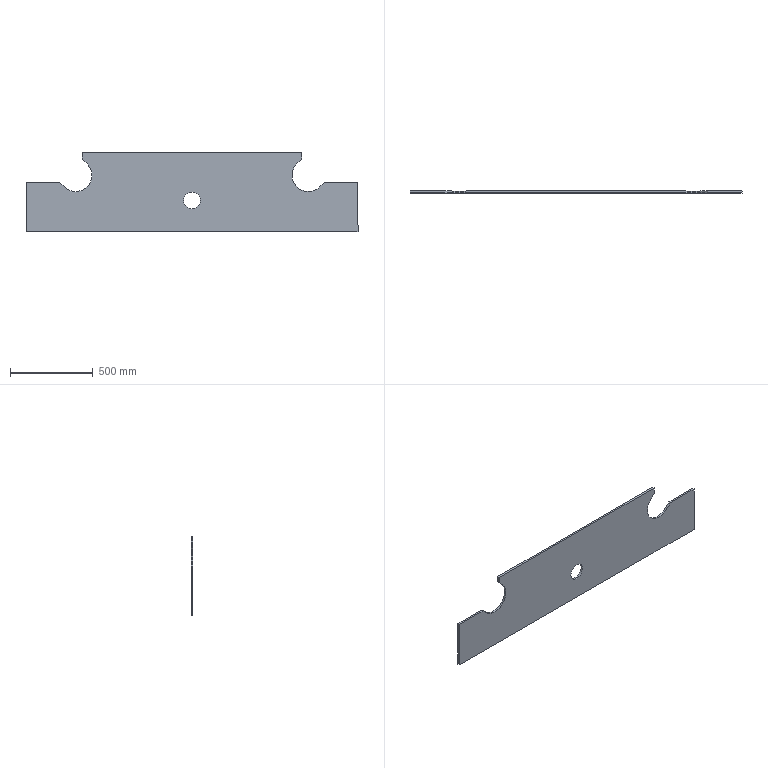Component | SolidWorks | SidePlate-2 | 1 solid | 19 faces | box 2000 x 12 x 476 mm | volume 9555406 mm3 | plane 14 | cylinder 5 | commonest cylinder face diameters 195 x3 100 x2 | material Plain Carbon Steel
STEP:
#1=COLOUR_RGB('',0.7922,0.8196,0.9333);
#2=FILL_AREA_STYLE_COLOUR('',#1);
#3=FILL_AREA_STYLE('',(#2));
#4=SURFACE_STYLE_FILL_AREA(#3);
#5=SURFACE_SIDE_STYLE('',(#4));
#6=SURFACE_STYLE_USAGE(.BOTH.,#5);
#7=PRESENTATION_STYLE_ASSIGNMENT((#6));
#8=CARTESIAN_POINT('',(51.204,45.014,72.956));
#9=VERTEX_POINT('',#8);
#10=CARTESIAN_POINT('',(47.267,45.014,72.956));
#11=VERTEX_POINT('',#10);
#12=CARTESIAN_POINT('',(49.235,45.014,72.956));
#13=DIRECTION('',(-0.,-1.,-0.));
#14=DIRECTION('',(-1.,0.,-0.));
#15=AXIS2_PLACEMENT_3D('',#12,#13,#14);
#16=CIRCLE('',#15,1.969);
#17=EDGE_CURVE('',#9,#11,#16,.T.);
#18=ORIENTED_EDGE('',*,*,#17,.F.);
#19=CARTESIAN_POINT('',(51.204,44.541,72.956));
#20=VERTEX_POINT('',#19);
#21=CARTESIAN_POINT('',(51.204,45.014,72.956));
#22=DIRECTION('',(-0.,-1.,-0.));
#23=VECTOR('',#22,39.37);
#24=LINE('',#21,#23);
#25=EDGE_CURVE('',#9,#20,#24,.T.);
#26=ORIENTED_EDGE('',*,*,#25,.T.);
#27=CARTESIAN_POINT('',(47.267,44.541,72.956));
#28=VERTEX_POINT('',#27);
#29=CARTESIAN_POINT('',(49.235,44.541,72.956));
#30=DIRECTION('',(-0.,-1.,-0.));
#31=DIRECTION('',(-1.,0.,-0.));
#32=AXIS2_PLACEMENT_3D('',#29,#30,#31);
#33=CIRCLE('',#32,1.969);
#34=EDGE_CURVE('',#20,#28,#33,.T.);
#35=ORIENTED_EDGE('',*,*,#34,.T.);
#36=CARTESIAN_POINT('',(47.267,45.014,72.956));
#37=DIRECTION('',(-0.,-1.,-0.));
#38=VECTOR('',#37,39.37);
#39=LINE('',#36,#38);
#40=EDGE_CURVE('',#11,#28,#39,.T.);
#41=ORIENTED_EDGE('',*,*,#40,.F.);
#42=EDGE_LOOP('',(#18,#26,#35,#41));
#43=FACE_OUTER_BOUND('',#42,.T.);
#44=CARTESIAN_POINT('',(49.235,45.014,72.956));
#45=DIRECTION('',(-0.,-1.,-0.));
#46=DIRECTION('',(-1.,0.,-0.));
#47=AXIS2_PLACEMENT_3D('',#44,#45,#46);
#48=CYLINDRICAL_SURFACE('',#47,1.969);
#49=ADVANCED_FACE('',(#43),#48,.F.);
#50=CARTESIAN_POINT('',(79.503,45.014,76.142));
#51=VERTEX_POINT('',#50);
#52=CARTESIAN_POINT('',(72.956,45.014,78.862));
#53=VERTEX_POINT('',#52);
#54=CARTESIAN_POINT('',(76.794,45.014,78.862));
#55=DIRECTION('',(0.,1.,0.));
#56=DIRECTION('',(1.,-0.,0.));
#57=AXIS2_PLACEMENT_3D('',#54,#55,#56);
#58=CIRCLE('',#57,3.839);
#59=EDGE_CURVE('',#51,#53,#58,.T.);
#60=ORIENTED_EDGE('',*,*,#59,.T.);
#61=CARTESIAN_POINT('',(72.956,44.541,78.862));
#62=VERTEX_POINT('',#61);
#63=CARTESIAN_POINT('',(72.956,45.014,78.862));
#64=DIRECTION('',(-0.,-1.,-0.));
#65=VECTOR('',#64,39.37);
#66=LINE('',#63,#65);
#67=EDGE_CURVE('',#53,#62,#66,.T.);
#68=ORIENTED_EDGE('',*,*,#67,.T.);
#69=CARTESIAN_POINT('',(79.503,44.541,76.142));
#70=VERTEX_POINT('',#69);
#71=CARTESIAN_POINT('',(76.794,44.541,78.862));
#72=DIRECTION('',(0.,1.,0.));
#73=DIRECTION('',(1.,-0.,0.));
#74=AXIS2_PLACEMENT_3D('',#71,#72,#73);
#75=CIRCLE('',#74,3.839);
#76=EDGE_CURVE('',#70,#62,#75,.T.);
#77=ORIENTED_EDGE('',*,*,#76,.F.);
#78=CARTESIAN_POINT('',(79.503,45.014,76.142));
#79=DIRECTION('',(-0.,-1.,-0.));
#80=VECTOR('',#79,39.37);
#81=LINE('',#78,#80);
#82=EDGE_CURVE('',#51,#70,#81,.T.);
#83=ORIENTED_EDGE('',*,*,#82,.F.);
#84=EDGE_LOOP('',(#60,#68,#77,#83));
#85=FACE_OUTER_BOUND('',#84,.T.);
#86=CARTESIAN_POINT('',(76.794,45.014,78.862));
#87=DIRECTION('',(-0.,-1.,-0.));
#88=DIRECTION('',(-1.,0.,-0.));
#89=AXIS2_PLACEMENT_3D('',#86,#87,#88);
#90=CYLINDRICAL_SURFACE('',#89,3.839);
#91=ADVANCED_FACE('',(#85),#90,.F.);
#92=CARTESIAN_POINT('',(88.605,44.541,65.555));
#93=VERTEX_POINT('',#92);
#94=CARTESIAN_POINT('',(88.605,44.541,77.287));
#95=VERTEX_POINT('',#94);
#96=CARTESIAN_POINT('',(88.605,44.541,65.555));
#97=DIRECTION('',(-0.,-0.,1.));
#98=VECTOR('',#97,39.37);
#99=LINE('',#96,#98);
#100=EDGE_CURVE('',#93,#95,#99,.T.);
#101=ORIENTED_EDGE('',*,*,#100,.F.);
#102=CARTESIAN_POINT('',(88.605,45.014,65.555));
#103=VERTEX_POINT('',#102);
#104=CARTESIAN_POINT('',(88.605,45.014,65.555));
#105=DIRECTION('',(-0.,-1.,-0.));
#106=VECTOR('',#105,39.37);
#107=LINE('',#104,#106);
#108=EDGE_CURVE('',#103,#93,#107,.T.);
#109=ORIENTED_EDGE('',*,*,#108,.F.);
#110=CARTESIAN_POINT('',(88.605,45.014,77.287));
#111=VERTEX_POINT('',#110);
#112=CARTESIAN_POINT('',(88.605,45.014,65.555));
#113=DIRECTION('',(-0.,-0.,1.));
#114=VECTOR('',#113,39.37);
#115=LINE('',#112,#114);
#116=EDGE_CURVE('',#103,#111,#115,.T.);
#117=ORIENTED_EDGE('',*,*,#116,.T.);
#118=CARTESIAN_POINT('',(88.605,45.014,77.287));
#119=DIRECTION('',(-0.,-1.,-0.));
#120=VECTOR('',#119,39.37);
#121=LINE('',#118,#120);
#122=EDGE_CURVE('',#111,#95,#121,.T.);
#123=ORIENTED_EDGE('',*,*,#122,.T.);
#124=EDGE_LOOP('',(#101,#109,#117,#123));
#125=FACE_OUTER_BOUND('',#124,.T.);
#126=CARTESIAN_POINT('',(88.605,45.014,65.555));
#127=DIRECTION('',(1.,-0.,0.));
#128=DIRECTION('',(-0.,-0.,1.));
#129=AXIS2_PLACEMENT_3D('',#126,#127,#128);
#130=PLANE('',#129);
#131=ADVANCED_FACE('',(#125),#130,.T.);
#132=CARTESIAN_POINT('',(9.865,44.541,65.555));
#133=VERTEX_POINT('',#132);
#134=CARTESIAN_POINT('',(88.605,44.541,65.555));
#135=DIRECTION('',(1.,-0.,0.));
#136=VECTOR('',#135,39.37);
#137=LINE('',#134,#136);
#138=EDGE_CURVE('',#133,#93,#137,.T.);
#139=ORIENTED_EDGE('',*,*,#138,.F.);
#140=CARTESIAN_POINT('',(9.865,45.014,65.555));
#141=VERTEX_POINT('',#140);
#142=CARTESIAN_POINT('',(9.865,45.014,65.555));
#143=DIRECTION('',(-0.,-1.,-0.));
#144=VECTOR('',#143,39.37);
#145=LINE('',#142,#144);
#146=EDGE_CURVE('',#141,#133,#145,.T.);
#147=ORIENTED_EDGE('',*,*,#146,.F.);
#148=CARTESIAN_POINT('',(88.605,45.014,65.555));
#149=DIRECTION('',(1.,-0.,0.));
#150=VECTOR('',#149,39.37);
#151=LINE('',#148,#150);
#152=EDGE_CURVE('',#141,#103,#151,.T.);
#153=ORIENTED_EDGE('',*,*,#152,.T.);
#154=ORIENTED_EDGE('',*,*,#108,.T.);
#155=EDGE_LOOP('',(#139,#147,#153,#154));
#156=FACE_OUTER_BOUND('',#155,.T.);
#157=CARTESIAN_POINT('',(88.605,45.014,65.555));
#158=DIRECTION('',(0.,0.,-1.));
#159=DIRECTION('',(1.,-0.,0.));
#160=AXIS2_PLACEMENT_3D('',#157,#158,#159);
#161=PLANE('',#160);
#162=ADVANCED_FACE('',(#156),#161,.T.);
#163=CARTESIAN_POINT('',(9.865,44.541,77.287));
#164=VERTEX_POINT('',#163);
#165=CARTESIAN_POINT('',(9.865,44.541,65.555));
#166=DIRECTION('',(0.,0.,-1.));
#167=VECTOR('',#166,39.37);
#168=LINE('',#165,#167);
#169=EDGE_CURVE('',#164,#133,#168,.T.);
#170=ORIENTED_EDGE('',*,*,#169,.F.);
#171=CARTESIAN_POINT('',(9.865,45.014,77.287));
#172=VERTEX_POINT('',#171);
#173=CARTESIAN_POINT('',(9.865,45.014,77.287));
#174=DIRECTION('',(-0.,-1.,-0.));
#175=VECTOR('',#174,39.37);
#176=LINE('',#173,#175);
#177=EDGE_CURVE('',#172,#164,#176,.T.);
#178=ORIENTED_EDGE('',*,*,#177,.F.);
#179=CARTESIAN_POINT('',(9.865,45.014,65.555));
#180=DIRECTION('',(0.,0.,-1.));
#181=VECTOR('',#180,39.37);
#182=LINE('',#179,#181);
#183=EDGE_CURVE('',#172,#141,#182,.T.);
#184=ORIENTED_EDGE('',*,*,#183,.T.);
#185=ORIENTED_EDGE('',*,*,#146,.T.);
#186=EDGE_LOOP('',(#170,#178,#184,#185));
#187=FACE_OUTER_BOUND('',#186,.T.);
#188=CARTESIAN_POINT('',(9.865,45.014,65.555));
#189=DIRECTION('',(-1.,0.,-0.));
#190=DIRECTION('',(0.,0.,-1.));
#191=AXIS2_PLACEMENT_3D('',#188,#189,#190);
#192=PLANE('',#191);
#193=ADVANCED_FACE('',(#187),#192,.T.);
#194=CARTESIAN_POINT('',(17.818,44.541,77.287));
#195=VERTEX_POINT('',#194);
#196=CARTESIAN_POINT('',(9.865,44.541,77.287));
#197=DIRECTION('',(-1.,0.,-0.));
#198=VECTOR('',#197,39.37);
#199=LINE('',#196,#198);
#200=EDGE_CURVE('',#195,#164,#199,.T.);
#201=ORIENTED_EDGE('',*,*,#200,.F.);
#202=CARTESIAN_POINT('',(17.818,45.014,77.287));
#203=VERTEX_POINT('',#202);
#204=CARTESIAN_POINT('',(17.818,45.014,77.287));
#205=DIRECTION('',(-0.,-1.,-0.));
#206=VECTOR('',#205,39.37);
#207=LINE('',#204,#206);
#208=EDGE_CURVE('',#203,#195,#207,.T.);
#209=ORIENTED_EDGE('',*,*,#208,.F.);
#210=CARTESIAN_POINT('',(9.865,45.014,77.287));
#211=DIRECTION('',(-1.,0.,-0.));
#212=VECTOR('',#211,39.37);
#213=LINE('',#210,#212);
#214=EDGE_CURVE('',#203,#172,#213,.T.);
#215=ORIENTED_EDGE('',*,*,#214,.T.);
#216=ORIENTED_EDGE('',*,*,#177,.T.);
#217=EDGE_LOOP('',(#201,#209,#215,#216));
#218=FACE_OUTER_BOUND('',#217,.T.);
#219=CARTESIAN_POINT('',(9.865,45.014,77.287));
#220=DIRECTION('',(-0.,-0.,1.));
#221=DIRECTION('',(-1.,0.,-0.));
#222=AXIS2_PLACEMENT_3D('',#219,#220,#221);
#223=PLANE('',#222);
#224=ADVANCED_FACE('',(#218),#223,.T.);
#225=CARTESIAN_POINT('',(18.967,44.541,76.142));
#226=VERTEX_POINT('',#225);
#227=CARTESIAN_POINT('',(17.818,44.541,77.287));
#228=DIRECTION('',(-0.7085,-0.,0.7057));
#229=VECTOR('',#228,39.37);
#230=LINE('',#227,#229);
#231=EDGE_CURVE('',#226,#195,#230,.T.);
#232=ORIENTED_EDGE('',*,*,#231,.F.);
#233=CARTESIAN_POINT('',(18.967,45.014,76.142));
#234=VERTEX_POINT('',#233);
#235=CARTESIAN_POINT('',(18.967,45.014,76.142));
#236=DIRECTION('',(-0.,-1.,-0.));
#237=VECTOR('',#236,39.37);
#238=LINE('',#235,#237);
#239=EDGE_CURVE('',#234,#226,#238,.T.);
#240=ORIENTED_EDGE('',*,*,#239,.F.);
#241=CARTESIAN_POINT('',(17.818,45.014,77.287));
#242=DIRECTION('',(-0.7085,-0.,0.7057));
#243=VECTOR('',#242,39.37);
#244=LINE('',#241,#243);
#245=EDGE_CURVE('',#234,#203,#244,.T.);
#246=ORIENTED_EDGE('',*,*,#245,.T.);
#247=ORIENTED_EDGE('',*,*,#208,.T.);
#248=EDGE_LOOP('',(#232,#240,#246,#247));
#249=FACE_OUTER_BOUND('',#248,.T.);
#250=CARTESIAN_POINT('',(17.818,45.014,77.287));
#251=DIRECTION('',(0.7057,-0.,0.7085));
#252=DIRECTION('',(-0.7085,-0.,0.7057));
#253=AXIS2_PLACEMENT_3D('',#250,#251,#252);
#254=PLANE('',#253);
#255=ADVANCED_FACE('',(#249),#254,.T.);
#256=CARTESIAN_POINT('',(24.396,44.541,81.571));
#257=VERTEX_POINT('',#256);
#258=CARTESIAN_POINT('',(21.676,44.541,78.862));
#259=DIRECTION('',(0.,1.,0.));
#260=DIRECTION('',(-1.,0.,-0.));
#261=AXIS2_PLACEMENT_3D('',#258,#259,#260);
#262=CIRCLE('',#261,3.839);
#263=EDGE_CURVE('',#257,#226,#262,.T.);
#264=ORIENTED_EDGE('',*,*,#263,.F.);
#265=CARTESIAN_POINT('',(24.396,45.014,81.571));
#266=VERTEX_POINT('',#265);
#267=CARTESIAN_POINT('',(24.396,45.014,81.571));
#268=DIRECTION('',(-0.,-1.,-0.));
#269=VECTOR('',#268,39.37);
#270=LINE('',#267,#269);
#271=EDGE_CURVE('',#266,#257,#270,.T.);
#272=ORIENTED_EDGE('',*,*,#271,.F.);
#273=CARTESIAN_POINT('',(21.676,45.014,78.862));
#274=DIRECTION('',(0.,1.,0.));
#275=DIRECTION('',(-1.,0.,-0.));
#276=AXIS2_PLACEMENT_3D('',#273,#274,#275);
#277=CIRCLE('',#276,3.839);
#278=EDGE_CURVE('',#266,#234,#277,.T.);
#279=ORIENTED_EDGE('',*,*,#278,.T.);
#280=ORIENTED_EDGE('',*,*,#239,.T.);
#281=EDGE_LOOP('',(#264,#272,#279,#280));
#282=FACE_OUTER_BOUND('',#281,.T.);
#283=CARTESIAN_POINT('',(21.676,45.014,78.862));
#284=DIRECTION('',(-0.,-1.,-0.));
#285=DIRECTION('',(-1.,0.,-0.));
#286=AXIS2_PLACEMENT_3D('',#283,#284,#285);
#287=CYLINDRICAL_SURFACE('',#286,3.839);
#288=ADVANCED_FACE('',(#282),#287,.F.);
#289=CARTESIAN_POINT('',(23.251,44.541,82.72));
#290=VERTEX_POINT('',#289);
#291=CARTESIAN_POINT('',(23.251,44.541,82.72));
#292=DIRECTION('',(0.7057,0.,-0.7085));
#293=VECTOR('',#292,39.37);
#294=LINE('',#291,#293);
#295=EDGE_CURVE('',#290,#257,#294,.T.);
#296=ORIENTED_EDGE('',*,*,#295,.F.);
#297=CARTESIAN_POINT('',(23.251,45.014,82.72));
#298=VERTEX_POINT('',#297);
#299=CARTESIAN_POINT('',(23.251,45.014,82.72));
#300=DIRECTION('',(-0.,-1.,-0.));
#301=VECTOR('',#300,39.37);
#302=LINE('',#299,#301);
#303=EDGE_CURVE('',#298,#290,#302,.T.);
#304=ORIENTED_EDGE('',*,*,#303,.F.);
#305=CARTESIAN_POINT('',(23.251,45.014,82.72));
#306=DIRECTION('',(0.7057,0.,-0.7085));
#307=VECTOR('',#306,39.37);
#308=LINE('',#305,#307);
#309=EDGE_CURVE('',#298,#266,#308,.T.);
#310=ORIENTED_EDGE('',*,*,#309,.T.);
#311=ORIENTED_EDGE('',*,*,#271,.T.);
#312=EDGE_LOOP('',(#296,#304,#310,#311));
#313=FACE_OUTER_BOUND('',#312,.T.);
#314=CARTESIAN_POINT('',(23.251,45.014,82.72));
#315=DIRECTION('',(-0.7085,0.,-0.7057));
#316=DIRECTION('',(0.7057,0.,-0.7085));
#317=AXIS2_PLACEMENT_3D('',#314,#315,#316);
#318=PLANE('',#317);
#319=ADVANCED_FACE('',(#313),#318,.T.);
#320=CARTESIAN_POINT('',(23.251,44.541,84.295));
#321=VERTEX_POINT('',#320);
#322=CARTESIAN_POINT('',(23.251,44.541,84.295));
#323=DIRECTION('',(0.,0.,-1.));
#324=VECTOR('',#323,39.37);
#325=LINE('',#322,#324);
#326=EDGE_CURVE('',#321,#290,#325,.T.);
#327=ORIENTED_EDGE('',*,*,#326,.F.);
#328=CARTESIAN_POINT('',(23.251,45.014,84.295));
#329=VERTEX_POINT('',#328);
#330=CARTESIAN_POINT('',(23.251,45.014,84.295));
#331=DIRECTION('',(-0.,-1.,-0.));
#332=VECTOR('',#331,39.37);
#333=LINE('',#330,#332);
#334=EDGE_CURVE('',#329,#321,#333,.T.);
#335=ORIENTED_EDGE('',*,*,#334,.F.);
#336=CARTESIAN_POINT('',(23.251,45.014,84.295));
#337=DIRECTION('',(0.,0.,-1.));
#338=VECTOR('',#337,39.37);
#339=LINE('',#336,#338);
#340=EDGE_CURVE('',#329,#298,#339,.T.);
#341=ORIENTED_EDGE('',*,*,#340,.T.);
#342=ORIENTED_EDGE('',*,*,#303,.T.);
#343=EDGE_LOOP('',(#327,#335,#341,#342));
#344=FACE_OUTER_BOUND('',#343,.T.);
#345=CARTESIAN_POINT('',(23.251,45.014,84.295));
#346=DIRECTION('',(-1.,0.,-0.));
#347=DIRECTION('',(0.,0.,-1.));
#348=AXIS2_PLACEMENT_3D('',#345,#346,#347);
#349=PLANE('',#348);
#350=ADVANCED_FACE('',(#344),#349,.T.);
#351=CARTESIAN_POINT('',(75.22,44.541,84.295));
#352=VERTEX_POINT('',#351);
#353=CARTESIAN_POINT('',(75.22,44.541,84.295));
#354=DIRECTION('',(-1.,0.,-0.));
#355=VECTOR('',#354,39.37);
#356=LINE('',#353,#355);
#357=EDGE_CURVE('',#352,#321,#356,.T.);
#358=ORIENTED_EDGE('',*,*,#357,.F.);
#359=CARTESIAN_POINT('',(75.22,45.014,84.295));
#360=VERTEX_POINT('',#359);
#361=CARTESIAN_POINT('',(75.22,45.014,84.295));
#362=DIRECTION('',(-0.,-1.,-0.));
#363=VECTOR('',#362,39.37);
#364=LINE('',#361,#363);
#365=EDGE_CURVE('',#360,#352,#364,.T.);
#366=ORIENTED_EDGE('',*,*,#365,.F.);
#367=CARTESIAN_POINT('',(75.22,45.014,84.295));
#368=DIRECTION('',(-1.,0.,-0.));
#369=VECTOR('',#368,39.37);
#370=LINE('',#367,#369);
#371=EDGE_CURVE('',#360,#329,#370,.T.);
#372=ORIENTED_EDGE('',*,*,#371,.T.);
#373=ORIENTED_EDGE('',*,*,#334,.T.);
#374=EDGE_LOOP('',(#358,#366,#372,#373));
#375=FACE_OUTER_BOUND('',#374,.T.);
#376=CARTESIAN_POINT('',(75.22,45.014,84.295));
#377=DIRECTION('',(-0.,-0.,1.));
#378=DIRECTION('',(-1.,0.,-0.));
#379=AXIS2_PLACEMENT_3D('',#376,#377,#378);
#380=PLANE('',#379);
#381=ADVANCED_FACE('',(#375),#380,.T.);
#382=CARTESIAN_POINT('',(75.22,44.541,82.72));
#383=VERTEX_POINT('',#382);
#384=CARTESIAN_POINT('',(75.22,44.541,84.295));
#385=DIRECTION('',(-0.,-0.,1.));
#386=VECTOR('',#385,39.37);
#387=LINE('',#384,#386);
#388=EDGE_CURVE('',#383,#352,#387,.T.);
#389=ORIENTED_EDGE('',*,*,#388,.F.);
#390=CARTESIAN_POINT('',(75.22,45.014,82.72));
#391=VERTEX_POINT('',#390);
#392=CARTESIAN_POINT('',(75.22,45.014,82.72));
#393=DIRECTION('',(-0.,-1.,-0.));
#394=VECTOR('',#393,39.37);
#395=LINE('',#392,#394);
#396=EDGE_CURVE('',#391,#383,#395,.T.);
#397=ORIENTED_EDGE('',*,*,#396,.F.);
#398=CARTESIAN_POINT('',(75.22,45.014,84.295));
#399=DIRECTION('',(-0.,-0.,1.));
#400=VECTOR('',#399,39.37);
#401=LINE('',#398,#400);
#402=EDGE_CURVE('',#391,#360,#401,.T.);
#403=ORIENTED_EDGE('',*,*,#402,.T.);
#404=ORIENTED_EDGE('',*,*,#365,.T.);
#405=EDGE_LOOP('',(#389,#397,#403,#404));
#406=FACE_OUTER_BOUND('',#405,.T.);
#407=CARTESIAN_POINT('',(75.22,45.014,84.295));
#408=DIRECTION('',(1.,-0.,0.));
#409=DIRECTION('',(-0.,-0.,1.));
#410=AXIS2_PLACEMENT_3D('',#407,#408,#409);
#411=PLANE('',#410);
#412=ADVANCED_FACE('',(#406),#411,.T.);
#413=CARTESIAN_POINT('',(74.075,44.541,81.571));
#414=VERTEX_POINT('',#413);
#415=CARTESIAN_POINT('',(75.22,44.541,82.72));
#416=DIRECTION('',(0.7057,-0.,0.7085));
#417=VECTOR('',#416,39.37);
#418=LINE('',#415,#417);
#419=EDGE_CURVE('',#414,#383,#418,.T.);
#420=ORIENTED_EDGE('',*,*,#419,.F.);
#421=CARTESIAN_POINT('',(74.075,45.014,81.571));
#422=VERTEX_POINT('',#421);
#423=CARTESIAN_POINT('',(74.075,45.014,81.571));
#424=DIRECTION('',(-0.,-1.,-0.));
#425=VECTOR('',#424,39.37);
#426=LINE('',#423,#425);
#427=EDGE_CURVE('',#422,#414,#426,.T.);
#428=ORIENTED_EDGE('',*,*,#427,.F.);
#429=CARTESIAN_POINT('',(75.22,45.014,82.72));
#430=DIRECTION('',(0.7057,-0.,0.7085));
#431=VECTOR('',#430,39.37);
#432=LINE('',#429,#431);
#433=EDGE_CURVE('',#422,#391,#432,.T.);
#434=ORIENTED_EDGE('',*,*,#433,.T.);
#435=ORIENTED_EDGE('',*,*,#396,.T.);
#436=EDGE_LOOP('',(#420,#428,#434,#435));
#437=FACE_OUTER_BOUND('',#436,.T.);
#438=CARTESIAN_POINT('',(75.22,45.014,82.72));
#439=DIRECTION('',(0.7085,0.,-0.7057));
#440=DIRECTION('',(0.7057,-0.,0.7085));
#441=AXIS2_PLACEMENT_3D('',#438,#439,#440);
#442=PLANE('',#441);
#443=ADVANCED_FACE('',(#437),#442,.T.);
#444=ORIENTED_EDGE('',*,*,#67,.F.);
#445=CARTESIAN_POINT('',(76.794,45.014,78.862));
#446=DIRECTION('',(0.,1.,0.));
#447=DIRECTION('',(1.,-0.,0.));
#448=AXIS2_PLACEMENT_3D('',#445,#446,#447);
#449=CIRCLE('',#448,3.839);
#450=EDGE_CURVE('',#53,#422,#449,.T.);
#451=ORIENTED_EDGE('',*,*,#450,.T.);
#452=ORIENTED_EDGE('',*,*,#427,.T.);
#453=CARTESIAN_POINT('',(76.794,44.541,78.862));
#454=DIRECTION('',(0.,1.,0.));
#455=DIRECTION('',(1.,-0.,0.));
#456=AXIS2_PLACEMENT_3D('',#453,#454,#455);
#457=CIRCLE('',#456,3.839);
#458=EDGE_CURVE('',#62,#414,#457,.T.);
#459=ORIENTED_EDGE('',*,*,#458,.F.);
#460=EDGE_LOOP('',(#444,#451,#452,#459));
#461=FACE_OUTER_BOUND('',#460,.T.);
#462=CARTESIAN_POINT('',(76.794,45.014,78.862));
#463=DIRECTION('',(-0.,-1.,-0.));
#464=DIRECTION('',(-1.,0.,-0.));
#465=AXIS2_PLACEMENT_3D('',#462,#463,#464);
#466=CYLINDRICAL_SURFACE('',#465,3.839);
#467=ADVANCED_FACE('',(#461),#466,.F.);
#468=CARTESIAN_POINT('',(80.653,44.541,77.287));
#469=VERTEX_POINT('',#468);
#470=CARTESIAN_POINT('',(80.653,44.541,77.287));
#471=DIRECTION('',(-0.7085,0.,-0.7057));
#472=VECTOR('',#471,39.37);
#473=LINE('',#470,#472);
#474=EDGE_CURVE('',#469,#70,#473,.T.);
#475=ORIENTED_EDGE('',*,*,#474,.F.);
#476=CARTESIAN_POINT('',(80.653,45.014,77.287));
#477=VERTEX_POINT('',#476);
#478=CARTESIAN_POINT('',(80.653,45.014,77.287));
#479=DIRECTION('',(-0.,-1.,-0.));
#480=VECTOR('',#479,39.37);
#481=LINE('',#478,#480);
#482=EDGE_CURVE('',#477,#469,#481,.T.);
#483=ORIENTED_EDGE('',*,*,#482,.F.);
#484=CARTESIAN_POINT('',(80.653,45.014,77.287));
#485=DIRECTION('',(-0.7085,0.,-0.7057));
#486=VECTOR('',#485,39.37);
#487=LINE('',#484,#486);
#488=EDGE_CURVE('',#477,#51,#487,.T.);
#489=ORIENTED_EDGE('',*,*,#488,.T.);
#490=ORIENTED_EDGE('',*,*,#82,.T.);
#491=EDGE_LOOP('',(#475,#483,#489,#490));
#492=FACE_OUTER_BOUND('',#491,.T.);
#493=CARTESIAN_POINT('',(80.653,45.014,77.287));
#494=DIRECTION('',(-0.7057,-0.,0.7085));
#495=DIRECTION('',(-0.7085,0.,-0.7057));
#496=AXIS2_PLACEMENT_3D('',#493,#494,#495);
#497=PLANE('',#496);
#498=ADVANCED_FACE('',(#492),#497,.T.);
#499=CARTESIAN_POINT('',(88.605,44.541,77.287));
#500=DIRECTION('',(-1.,0.,-0.));
#501=VECTOR('',#500,39.37);
#502=LINE('',#499,#501);
#503=EDGE_CURVE('',#95,#469,#502,.T.);
#504=ORIENTED_EDGE('',*,*,#503,.F.);
#505=ORIENTED_EDGE('',*,*,#122,.F.);
#506=CARTESIAN_POINT('',(88.605,45.014,77.287));
#507=DIRECTION('',(-1.,0.,-0.));
#508=VECTOR('',#507,39.37);
#509=LINE('',#506,#508);
#510=EDGE_CURVE('',#111,#477,#509,.T.);
#511=ORIENTED_EDGE('',*,*,#510,.T.);
#512=ORIENTED_EDGE('',*,*,#482,.T.);
#513=EDGE_LOOP('',(#504,#505,#511,#512));
#514=FACE_OUTER_BOUND('',#513,.T.);
#515=CARTESIAN_POINT('',(88.605,45.014,77.287));
#516=DIRECTION('',(-0.,-0.,1.));
#517=DIRECTION('',(-1.,0.,-0.));
#518=AXIS2_PLACEMENT_3D('',#515,#516,#517);
#519=PLANE('',#518);
#520=ADVANCED_FACE('',(#514),#519,.T.);
#521=CARTESIAN_POINT('',(49.235,45.014,72.956));
#522=DIRECTION('',(-0.,-1.,-0.));
#523=DIRECTION('',(-1.,0.,-0.));
#524=AXIS2_PLACEMENT_3D('',#521,#522,#523);
#525=CIRCLE('',#524,1.969);
#526=EDGE_CURVE('',#11,#9,#525,.T.);
#527=ORIENTED_EDGE('',*,*,#526,.T.);
#528=ORIENTED_EDGE('',*,*,#17,.T.);
#529=EDGE_LOOP('',(#527,#528));
#530=FACE_BOUND('',#529,.T.);
#531=ORIENTED_EDGE('',*,*,#116,.F.);
#532=ORIENTED_EDGE('',*,*,#152,.F.);
#533=ORIENTED_EDGE('',*,*,#183,.F.);
#534=ORIENTED_EDGE('',*,*,#214,.F.);
#535=ORIENTED_EDGE('',*,*,#245,.F.);
#536=ORIENTED_EDGE('',*,*,#278,.F.);
#537=ORIENTED_EDGE('',*,*,#309,.F.);
#538=ORIENTED_EDGE('',*,*,#340,.F.);
#539=ORIENTED_EDGE('',*,*,#371,.F.);
#540=ORIENTED_EDGE('',*,*,#402,.F.);
#541=ORIENTED_EDGE('',*,*,#433,.F.);
#542=ORIENTED_EDGE('',*,*,#450,.F.);
#543=ORIENTED_EDGE('',*,*,#59,.F.);
#544=ORIENTED_EDGE('',*,*,#488,.F.);
#545=ORIENTED_EDGE('',*,*,#510,.F.);
#546=EDGE_LOOP('',(#531,#532,#533,#534,#535,#536,#537,#538,#539,#540,#541,#542,#543,#544,#545));
#547=FACE_OUTER_BOUND('',#546,.T.);
#548=CARTESIAN_POINT('',(76.794,45.014,78.862));
#549=DIRECTION('',(0.,1.,0.));
#550=DIRECTION('',(1.,-0.,0.));
#551=AXIS2_PLACEMENT_3D('',#548,#549,#550);
#552=PLANE('',#551);
#553=ADVANCED_FACE('',(#530,#547),#552,.T.);
#554=CARTESIAN_POINT('',(49.235,44.541,72.956));
#555=DIRECTION('',(-0.,-1.,-0.));
#556=DIRECTION('',(-1.,0.,-0.));
#557=AXIS2_PLACEMENT_3D('',#554,#555,#556);
#558=CIRCLE('',#557,1.969);
#559=EDGE_CURVE('',#28,#20,#558,.T.);
#560=ORIENTED_EDGE('',*,*,#559,.F.);
#561=ORIENTED_EDGE('',*,*,#34,.F.);
#562=EDGE_LOOP('',(#560,#561));
#563=FACE_BOUND('',#562,.T.);
#564=ORIENTED_EDGE('',*,*,#100,.T.);
#565=ORIENTED_EDGE('',*,*,#503,.T.);
#566=ORIENTED_EDGE('',*,*,#474,.T.);
#567=ORIENTED_EDGE('',*,*,#76,.T.);
#568=ORIENTED_EDGE('',*,*,#458,.T.);
#569=ORIENTED_EDGE('',*,*,#419,.T.);
#570=ORIENTED_EDGE('',*,*,#388,.T.);
#571=ORIENTED_EDGE('',*,*,#357,.T.);
#572=ORIENTED_EDGE('',*,*,#326,.T.);
#573=ORIENTED_EDGE('',*,*,#295,.T.);
#574=ORIENTED_EDGE('',*,*,#263,.T.);
#575=ORIENTED_EDGE('',*,*,#231,.T.);
#576=ORIENTED_EDGE('',*,*,#200,.T.);
#577=ORIENTED_EDGE('',*,*,#169,.T.);
#578=ORIENTED_EDGE('',*,*,#138,.T.);
#579=EDGE_LOOP('',(#564,#565,#566,#567,#568,#569,#570,#571,#572,#573,#574,#575,#576,#577,#578));
#580=FACE_OUTER_BOUND('',#579,.T.);
#581=CARTESIAN_POINT('',(76.794,44.541,78.862));
#582=DIRECTION('',(0.,1.,0.));
#583=DIRECTION('',(1.,-0.,0.));
#584=AXIS2_PLACEMENT_3D('',#581,#582,#583);
#585=PLANE('',#584);
#586=ADVANCED_FACE('',(#563,#580),#585,.F.);
#587=ORIENTED_EDGE('',*,*,#25,.F.);
#588=ORIENTED_EDGE('',*,*,#526,.F.);
#589=ORIENTED_EDGE('',*,*,#40,.T.);
#590=ORIENTED_EDGE('',*,*,#559,.T.);
#591=EDGE_LOOP('',(#587,#588,#589,#590));
#592=FACE_OUTER_BOUND('',#591,.T.);
#593=CARTESIAN_POINT('',(49.235,45.014,72.956));
#594=DIRECTION('',(-0.,-1.,-0.));
#595=DIRECTION('',(-1.,0.,-0.));
#596=AXIS2_PLACEMENT_3D('',#593,#594,#595);
#597=CYLINDRICAL_SURFACE('',#596,1.969);
#598=ADVANCED_FACE('',(#592),#597,.F.);
#599=CLOSED_SHELL('',(#49,#91,#131,#162,#193,#224,#255,#288,#319,#350,#381,#412,#443,#467,#498,#520,#553,#586,#598));
#600=MANIFOLD_SOLID_BREP('',#599);
#601=STYLED_ITEM('',(#7),#600);
#602=(LENGTH_UNIT()NAMED_UNIT(*)SI_UNIT($,.METRE.));
#603=LENGTH_MEASURE_WITH_UNIT(LENGTH_MEASURE(0.0254),#602);
#604=DIMENSIONAL_EXPONENTS(1.,0.,0.,0.,0.,0.,0.);
#605=(CONVERSION_BASED_UNIT('',#603)LENGTH_UNIT()NAMED_UNIT(#604));
#606=UNCERTAINTY_MEASURE_WITH_UNIT(LENGTH_MEASURE(0.00001),#605,'','');
#607=(NAMED_UNIT(*)PLANE_ANGLE_UNIT()SI_UNIT($,.RADIAN.));
#608=(NAMED_UNIT(*)SI_UNIT($,.STERADIAN.)SOLID_ANGLE_UNIT());
#609=(GEOMETRIC_REPRESENTATION_CONTEXT(3)GLOBAL_UNCERTAINTY_ASSIGNED_CONTEXT((#606))GLOBAL_UNIT_ASSIGNED_CONTEXT((#605,#607,#608))REPRESENTATION_CONTEXT('',''));
#610=MECHANICAL_DESIGN_GEOMETRIC_PRESENTATION_REPRESENTATION('',(#601),#609);
#611=CARTESIAN_POINT('',(0.,0.,0.));
#612=DIRECTION('',(0.,0.,1.));
#613=DIRECTION('',(1.,0.,0.));
#614=AXIS2_PLACEMENT_3D('',#611,#612,#613);
#615=(LENGTH_UNIT()NAMED_UNIT(*)SI_UNIT($,.METRE.));
#616=LENGTH_MEASURE_WITH_UNIT(LENGTH_MEASURE(0.0254),#615);
#617=DIMENSIONAL_EXPONENTS(1.,0.,0.,0.,0.,0.,0.);
#618=(CONVERSION_BASED_UNIT('',#616)LENGTH_UNIT()NAMED_UNIT(#617));
#619=UNCERTAINTY_MEASURE_WITH_UNIT(LENGTH_MEASURE(0.00001),#618,'','');
#620=(NAMED_UNIT(*)PLANE_ANGLE_UNIT()SI_UNIT($,.RADIAN.));
#621=(NAMED_UNIT(*)SI_UNIT($,.STERADIAN.)SOLID_ANGLE_UNIT());
#622=(GEOMETRIC_REPRESENTATION_CONTEXT(3)GLOBAL_UNCERTAINTY_ASSIGNED_CONTEXT((#619))GLOBAL_UNIT_ASSIGNED_CONTEXT((#618,#620,#621))REPRESENTATION_CONTEXT('',''));
#623=ADVANCED_BREP_SHAPE_REPRESENTATION('',(#600,#614),#622);
#624=PRESENTATION_LAYER_ASSIGNMENT('','',(#601));